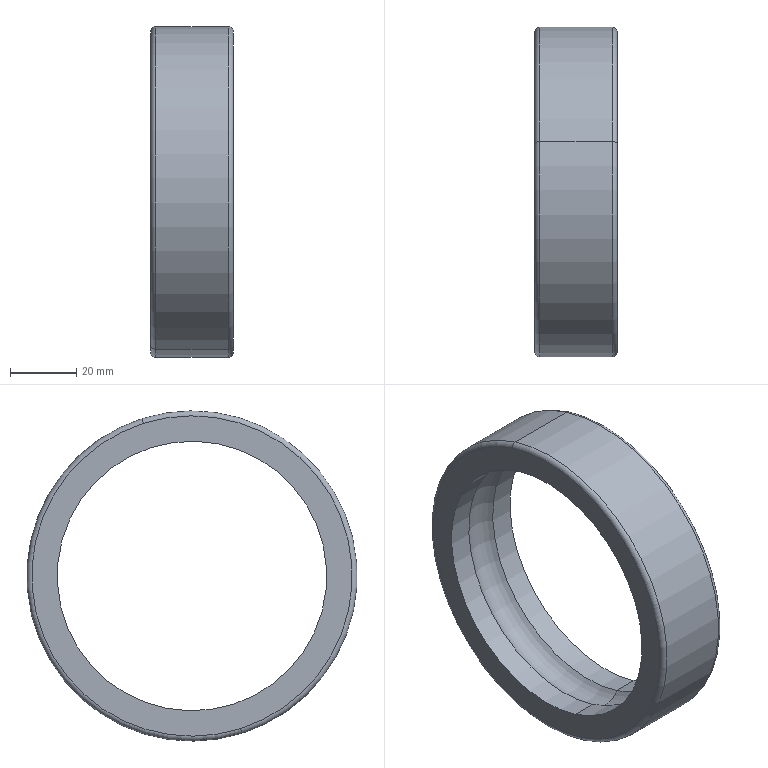Component | SolidWorks | UpperHousingAssembly-1_WormAxisAssembly-1_DeepGrooveBallBearing6309-1_BearingOuterRing-1 | 1 solid | 14 faces | box 25 x 100 x 100 mm | volume 61028 mm3 | torus 6 | cylinder 6 | plane 2 | commonest cylinder face diameters 81.6 x4 100 x2
build123d program:
from build123d import *

# Parameters (mm, degrees)
FILLET1_R = 1.5


with BuildPart() as part:
    # Sketch1 → Revolve1 (revolve)
    with BuildSketch(Plane.XY, mode=Mode.PRIVATE) as revolve1_sk:
        with BuildLine():
            Line((5.121, 40.8), (12.5, 40.8))
            Line((12.5, 40.8), (12.5, 50))
            Line((12.5, 50), (-12.5, 50))
            Line((-12.5, 50), (-12.5, 40.8))
            Line((-12.5, 40.8), (-5.121, 40.8))
            ThreePointArc((-5.121, 40.8), (0, 43.1), (5.121, 40.8))
        make_face()
    revolve(revolve1_sk.sketch.rotate(Axis((-5.851, 0, 0), (1, 0, 0)), 90), axis=Axis((-5.851, 0, 0), (1, 0, 0)))

    # Fillet1
    fillet1_edges = [part.edges().sort_by_distance(p)[0] for p in [
        (-12.5, 0, -50),
        (12.5, 0, -50),
    ]]
    fillet(fillet1_edges, radius=FILLET1_R)


solid = part.part

# Placed as in the assembly
solid = solid.moved(Location((1019.077, 1408.591, 1694.217), (0, 0, 0)))
STEP:
#1=CARTESIAN_POINT('',(40.613,54.879,64.881));
#2=VERTEX_POINT('',#1);
#3=CARTESIAN_POINT('',(40.613,56.034,68.522));
#4=VERTEX_POINT('',#3);
#5=CARTESIAN_POINT('',(40.613,55.456,66.701));
#6=DIRECTION('',(1.,0.,0.));
#7=DIRECTION('',(0.,0.3024,0.9532));
#8=AXIS2_PLACEMENT_3D('',#5,#6,#7);
#9=CIRCLE('',#8,1.909);
#10=EDGE_CURVE('',#2,#4,#9,.T.);
#11=ORIENTED_EDGE('',*,*,#10,.F.);
#12=CARTESIAN_POINT('',(40.554,54.861,64.825));
#13=VERTEX_POINT('',#12);
#14=CARTESIAN_POINT('',(40.554,54.879,64.881));
#15=DIRECTION('',(0.,0.9532,-0.3024));
#16=DIRECTION('',(0.,0.3024,0.9532));
#17=AXIS2_PLACEMENT_3D('',#14,#15,#16);
#18=CIRCLE('',#17,0.05906);
#19=EDGE_CURVE('',#2,#13,#18,.T.);
#20=ORIENTED_EDGE('',*,*,#19,.T.);
#21=CARTESIAN_POINT('',(40.554,56.052,68.578));
#22=VERTEX_POINT('',#21);
#23=CARTESIAN_POINT('',(40.554,55.456,66.701));
#24=DIRECTION('',(-1.,0.,0.));
#25=DIRECTION('',(0.,0.3024,0.9532));
#26=AXIS2_PLACEMENT_3D('',#23,#24,#25);
#27=CIRCLE('',#26,1.969);
#28=EDGE_CURVE('',#22,#13,#27,.T.);
#29=ORIENTED_EDGE('',*,*,#28,.F.);
#30=CARTESIAN_POINT('',(40.554,56.034,68.522));
#31=DIRECTION('',(0.,-0.9532,0.3024));
#32=DIRECTION('',(0.,-0.3024,-0.9532));
#33=AXIS2_PLACEMENT_3D('',#30,#31,#32);
#34=CIRCLE('',#33,0.05906);
#35=EDGE_CURVE('',#4,#22,#34,.T.);
#36=ORIENTED_EDGE('',*,*,#35,.F.);
#37=EDGE_LOOP('',(#11,#20,#29,#36));
#38=FACE_OUTER_BOUND('',#37,.T.);
#39=CARTESIAN_POINT('',(40.554,55.456,66.701));
#40=DIRECTION('',(-1.,0.,0.));
#41=DIRECTION('',(0.,0.3024,0.9532));
#42=AXIS2_PLACEMENT_3D('',#39,#40,#41);
#43=TOROIDAL_SURFACE('',#42,1.909,0.05906);
#44=ADVANCED_FACE('',(#38),#43,.T.);
#45=CARTESIAN_POINT('',(39.629,56.034,68.522));
#46=VERTEX_POINT('',#45);
#47=CARTESIAN_POINT('',(39.629,54.879,64.881));
#48=VERTEX_POINT('',#47);
#49=CARTESIAN_POINT('',(39.629,55.456,66.701));
#50=DIRECTION('',(-1.,0.,0.));
#51=DIRECTION('',(0.,-0.3024,-0.9532));
#52=AXIS2_PLACEMENT_3D('',#49,#50,#51);
#53=CIRCLE('',#52,1.909);
#54=EDGE_CURVE('',#46,#48,#53,.T.);
#55=ORIENTED_EDGE('',*,*,#54,.F.);
#56=CARTESIAN_POINT('',(39.688,56.052,68.578));
#57=VERTEX_POINT('',#56);
#58=CARTESIAN_POINT('',(39.688,56.034,68.522));
#59=DIRECTION('',(0.,0.9532,-0.3024));
#60=DIRECTION('',(0.,0.3024,0.9532));
#61=AXIS2_PLACEMENT_3D('',#58,#59,#60);
#62=CIRCLE('',#61,0.05906);
#63=EDGE_CURVE('',#46,#57,#62,.T.);
#64=ORIENTED_EDGE('',*,*,#63,.T.);
#65=CARTESIAN_POINT('',(39.688,54.861,64.825));
#66=VERTEX_POINT('',#65);
#67=CARTESIAN_POINT('',(39.688,55.456,66.701));
#68=DIRECTION('',(1.,0.,0.));
#69=DIRECTION('',(0.,-0.3024,-0.9532));
#70=AXIS2_PLACEMENT_3D('',#67,#68,#69);
#71=CIRCLE('',#70,1.969);
#72=EDGE_CURVE('',#66,#57,#71,.T.);
#73=ORIENTED_EDGE('',*,*,#72,.F.);
#74=CARTESIAN_POINT('',(39.688,54.879,64.881));
#75=DIRECTION('',(0.,-0.9532,0.3024));
#76=DIRECTION('',(0.,-0.3024,-0.9532));
#77=AXIS2_PLACEMENT_3D('',#74,#75,#76);
#78=CIRCLE('',#77,0.05906);
#79=EDGE_CURVE('',#48,#66,#78,.T.);
#80=ORIENTED_EDGE('',*,*,#79,.F.);
#81=EDGE_LOOP('',(#55,#64,#73,#80));
#82=FACE_OUTER_BOUND('',#81,.T.);
#83=CARTESIAN_POINT('',(39.688,55.456,66.701));
#84=DIRECTION('',(1.,0.,0.));
#85=DIRECTION('',(0.,-0.3024,-0.9532));
#86=AXIS2_PLACEMENT_3D('',#83,#84,#85);
#87=TOROIDAL_SURFACE('',#86,1.909,0.05906);
#88=ADVANCED_FACE('',(#82),#87,.T.);
#89=CARTESIAN_POINT('',(40.613,54.971,65.17));
#90=VERTEX_POINT('',#89);
#91=CARTESIAN_POINT('',(40.613,55.942,68.233));
#92=VERTEX_POINT('',#91);
#93=CARTESIAN_POINT('',(40.613,55.456,66.701));
#94=DIRECTION('',(-1.,0.,0.));
#95=DIRECTION('',(0.,0.3024,0.9532));
#96=AXIS2_PLACEMENT_3D('',#93,#94,#95);
#97=CIRCLE('',#96,1.606);
#98=EDGE_CURVE('',#90,#92,#97,.T.);
#99=ORIENTED_EDGE('',*,*,#98,.F.);
#100=CARTESIAN_POINT('',(40.323,54.971,65.17));
#101=VERTEX_POINT('',#100);
#102=CARTESIAN_POINT('',(39.891,54.971,65.17));
#103=DIRECTION('',(-1.,0.,0.));
#104=VECTOR('',#103,39.37);
#105=LINE('',#102,#104);
#106=EDGE_CURVE('',#90,#101,#105,.T.);
#107=ORIENTED_EDGE('',*,*,#106,.T.);
#108=CARTESIAN_POINT('',(40.323,55.942,68.233));
#109=VERTEX_POINT('',#108);
#110=CARTESIAN_POINT('',(40.323,55.456,66.701));
#111=DIRECTION('',(-1.,0.,0.));
#112=DIRECTION('',(0.,0.3024,0.9532));
#113=AXIS2_PLACEMENT_3D('',#110,#111,#112);
#114=CIRCLE('',#113,1.606);
#115=EDGE_CURVE('',#101,#109,#114,.T.);
#116=ORIENTED_EDGE('',*,*,#115,.T.);
#117=CARTESIAN_POINT('',(39.891,55.942,68.233));
#118=DIRECTION('',(-1.,0.,0.));
#119=VECTOR('',#118,39.37);
#120=LINE('',#117,#119);
#121=EDGE_CURVE('',#92,#109,#120,.T.);
#122=ORIENTED_EDGE('',*,*,#121,.F.);
#123=EDGE_LOOP('',(#99,#107,#116,#122));
#124=FACE_OUTER_BOUND('',#123,.T.);
#125=CARTESIAN_POINT('',(39.891,55.456,66.701));
#126=DIRECTION('',(-1.,0.,0.));
#127=DIRECTION('',(0.,0.3024,0.9532));
#128=AXIS2_PLACEMENT_3D('',#125,#126,#127);
#129=CYLINDRICAL_SURFACE('',#128,1.606);
#130=ADVANCED_FACE('',(#124),#129,.F.);
#131=ORIENTED_EDGE('',*,*,#115,.F.);
#132=CARTESIAN_POINT('',(39.92,54.971,65.17));
#133=VERTEX_POINT('',#132);
#134=CARTESIAN_POINT('',(40.121,55.025,65.341));
#135=DIRECTION('',(0.,0.9532,-0.3024));
#136=DIRECTION('',(0.,0.3024,0.9532));
#137=AXIS2_PLACEMENT_3D('',#134,#135,#136);
#138=CIRCLE('',#137,0.2697);
#139=EDGE_CURVE('',#101,#133,#138,.T.);
#140=ORIENTED_EDGE('',*,*,#139,.T.);
#141=CARTESIAN_POINT('',(39.92,55.942,68.233));
#142=VERTEX_POINT('',#141);
#143=CARTESIAN_POINT('',(39.92,55.456,66.701));
#144=DIRECTION('',(-1.,0.,0.));
#145=DIRECTION('',(0.,0.3024,0.9532));
#146=AXIS2_PLACEMENT_3D('',#143,#144,#145);
#147=CIRCLE('',#146,1.606);
#148=EDGE_CURVE('',#133,#142,#147,.T.);
#149=ORIENTED_EDGE('',*,*,#148,.T.);
#150=CARTESIAN_POINT('',(40.121,55.888,68.062));
#151=DIRECTION('',(0.,-0.9532,0.3024));
#152=DIRECTION('',(0.,-0.3024,-0.9532));
#153=AXIS2_PLACEMENT_3D('',#150,#151,#152);
#154=CIRCLE('',#153,0.2697);
#155=EDGE_CURVE('',#109,#142,#154,.T.);
#156=ORIENTED_EDGE('',*,*,#155,.F.);
#157=EDGE_LOOP('',(#131,#140,#149,#156));
#158=FACE_OUTER_BOUND('',#157,.T.);
#159=CARTESIAN_POINT('',(40.121,55.456,66.701));
#160=DIRECTION('',(-1.,0.,0.));
#161=DIRECTION('',(0.,0.3024,0.9532));
#162=AXIS2_PLACEMENT_3D('',#159,#160,#161);
#163=TOROIDAL_SURFACE('',#162,1.427,0.2697);
#164=ADVANCED_FACE('',(#158),#163,.F.);
#165=ORIENTED_EDGE('',*,*,#148,.F.);
#166=CARTESIAN_POINT('',(39.629,54.971,65.17));
#167=VERTEX_POINT('',#166);
#168=CARTESIAN_POINT('',(39.891,54.971,65.17));
#169=DIRECTION('',(-1.,0.,0.));
#170=VECTOR('',#169,39.37);
#171=LINE('',#168,#170);
#172=EDGE_CURVE('',#133,#167,#171,.T.);
#173=ORIENTED_EDGE('',*,*,#172,.T.);
#174=CARTESIAN_POINT('',(39.629,55.942,68.233));
#175=VERTEX_POINT('',#174);
#176=CARTESIAN_POINT('',(39.629,55.456,66.701));
#177=DIRECTION('',(-1.,0.,0.));
#178=DIRECTION('',(0.,0.3024,0.9532));
#179=AXIS2_PLACEMENT_3D('',#176,#177,#178);
#180=CIRCLE('',#179,1.606);
#181=EDGE_CURVE('',#167,#175,#180,.T.);
#182=ORIENTED_EDGE('',*,*,#181,.T.);
#183=CARTESIAN_POINT('',(39.891,55.942,68.233));
#184=DIRECTION('',(-1.,0.,0.));
#185=VECTOR('',#184,39.37);
#186=LINE('',#183,#185);
#187=EDGE_CURVE('',#142,#175,#186,.T.);
#188=ORIENTED_EDGE('',*,*,#187,.F.);
#189=EDGE_LOOP('',(#165,#173,#182,#188));
#190=FACE_OUTER_BOUND('',#189,.T.);
#191=CARTESIAN_POINT('',(39.891,55.456,66.701));
#192=DIRECTION('',(-1.,0.,0.));
#193=DIRECTION('',(0.,0.3024,0.9532));
#194=AXIS2_PLACEMENT_3D('',#191,#192,#193);
#195=CYLINDRICAL_SURFACE('',#194,1.606);
#196=ADVANCED_FACE('',(#190),#195,.F.);
#197=ORIENTED_EDGE('',*,*,#28,.T.);
#198=CARTESIAN_POINT('',(39.891,54.861,64.825));
#199=DIRECTION('',(-1.,0.,0.));
#200=VECTOR('',#199,39.37);
#201=LINE('',#198,#200);
#202=EDGE_CURVE('',#13,#66,#201,.T.);
#203=ORIENTED_EDGE('',*,*,#202,.T.);
#204=ORIENTED_EDGE('',*,*,#72,.T.);
#205=CARTESIAN_POINT('',(39.891,56.052,68.578));
#206=DIRECTION('',(-1.,0.,0.));
#207=VECTOR('',#206,39.37);
#208=LINE('',#205,#207);
#209=EDGE_CURVE('',#22,#57,#208,.T.);
#210=ORIENTED_EDGE('',*,*,#209,.F.);
#211=EDGE_LOOP('',(#197,#203,#204,#210));
#212=FACE_OUTER_BOUND('',#211,.T.);
#213=CARTESIAN_POINT('',(39.891,55.456,66.701));
#214=DIRECTION('',(-1.,0.,0.));
#215=DIRECTION('',(0.,0.3024,0.9532));
#216=AXIS2_PLACEMENT_3D('',#213,#214,#215);
#217=CYLINDRICAL_SURFACE('',#216,1.969);
#218=ADVANCED_FACE('',(#212),#217,.T.);
#219=CARTESIAN_POINT('',(40.613,55.456,66.701));
#220=DIRECTION('',(1.,0.,0.));
#221=DIRECTION('',(0.,0.3024,0.9532));
#222=AXIS2_PLACEMENT_3D('',#219,#220,#221);
#223=CIRCLE('',#222,1.909);
#224=EDGE_CURVE('',#4,#2,#223,.T.);
#225=ORIENTED_EDGE('',*,*,#224,.T.);
#226=ORIENTED_EDGE('',*,*,#10,.T.);
#227=EDGE_LOOP('',(#225,#226));
#228=FACE_OUTER_BOUND('',#227,.T.);
#229=CARTESIAN_POINT('',(40.613,55.456,66.701));
#230=DIRECTION('',(-1.,0.,0.));
#231=DIRECTION('',(0.,0.3024,0.9532));
#232=AXIS2_PLACEMENT_3D('',#229,#230,#231);
#233=CIRCLE('',#232,1.606);
#234=EDGE_CURVE('',#92,#90,#233,.T.);
#235=ORIENTED_EDGE('',*,*,#234,.T.);
#236=ORIENTED_EDGE('',*,*,#98,.T.);
#237=EDGE_LOOP('',(#235,#236));
#238=FACE_BOUND('',#237,.T.);
#239=CARTESIAN_POINT('',(40.613,57.333,66.106));
#240=DIRECTION('',(-1.,0.,0.));
#241=DIRECTION('',(0.,0.3024,0.9532));
#242=AXIS2_PLACEMENT_3D('',#239,#240,#241);
#243=PLANE('',#242);
#244=ADVANCED_FACE('',(#228,#238),#243,.F.);
#245=ORIENTED_EDGE('',*,*,#202,.F.);
#246=CARTESIAN_POINT('',(40.554,55.456,66.701));
#247=DIRECTION('',(-1.,0.,0.));
#248=DIRECTION('',(0.,0.3024,0.9532));
#249=AXIS2_PLACEMENT_3D('',#246,#247,#248);
#250=CIRCLE('',#249,1.969);
#251=EDGE_CURVE('',#13,#22,#250,.T.);
#252=ORIENTED_EDGE('',*,*,#251,.T.);
#253=ORIENTED_EDGE('',*,*,#209,.T.);
#254=CARTESIAN_POINT('',(39.688,55.456,66.701));
#255=DIRECTION('',(1.,0.,0.));
#256=DIRECTION('',(0.,-0.3024,-0.9532));
#257=AXIS2_PLACEMENT_3D('',#254,#255,#256);
#258=CIRCLE('',#257,1.969);
#259=EDGE_CURVE('',#57,#66,#258,.T.);
#260=ORIENTED_EDGE('',*,*,#259,.T.);
#261=EDGE_LOOP('',(#245,#252,#253,#260));
#262=FACE_OUTER_BOUND('',#261,.T.);
#263=CARTESIAN_POINT('',(39.891,55.456,66.701));
#264=DIRECTION('',(-1.,0.,0.));
#265=DIRECTION('',(0.,0.3024,0.9532));
#266=AXIS2_PLACEMENT_3D('',#263,#264,#265);
#267=CYLINDRICAL_SURFACE('',#266,1.969);
#268=ADVANCED_FACE('',(#262),#267,.T.);
#269=CARTESIAN_POINT('',(39.629,55.456,66.701));
#270=DIRECTION('',(-1.,0.,0.));
#271=DIRECTION('',(0.,-0.3024,-0.9532));
#272=AXIS2_PLACEMENT_3D('',#269,#270,#271);
#273=CIRCLE('',#272,1.909);
#274=EDGE_CURVE('',#48,#46,#273,.T.);
#275=ORIENTED_EDGE('',*,*,#274,.T.);
#276=ORIENTED_EDGE('',*,*,#54,.T.);
#277=EDGE_LOOP('',(#275,#276));
#278=FACE_OUTER_BOUND('',#277,.T.);
#279=CARTESIAN_POINT('',(39.629,55.456,66.701));
#280=DIRECTION('',(-1.,0.,0.));
#281=DIRECTION('',(0.,0.3024,0.9532));
#282=AXIS2_PLACEMENT_3D('',#279,#280,#281);
#283=CIRCLE('',#282,1.606);
#284=EDGE_CURVE('',#175,#167,#283,.T.);
#285=ORIENTED_EDGE('',*,*,#284,.F.);
#286=ORIENTED_EDGE('',*,*,#181,.F.);
#287=EDGE_LOOP('',(#285,#286));
#288=FACE_BOUND('',#287,.T.);
#289=CARTESIAN_POINT('',(39.629,57.333,66.106));
#290=DIRECTION('',(1.,0.,0.));
#291=DIRECTION('',(0.,-0.3024,-0.9532));
#292=AXIS2_PLACEMENT_3D('',#289,#290,#291);
#293=PLANE('',#292);
#294=ADVANCED_FACE('',(#278,#288),#293,.F.);
#295=ORIENTED_EDGE('',*,*,#172,.F.);
#296=CARTESIAN_POINT('',(39.92,55.456,66.701));
#297=DIRECTION('',(-1.,0.,0.));
#298=DIRECTION('',(0.,0.3024,0.9532));
#299=AXIS2_PLACEMENT_3D('',#296,#297,#298);
#300=CIRCLE('',#299,1.606);
#301=EDGE_CURVE('',#142,#133,#300,.T.);
#302=ORIENTED_EDGE('',*,*,#301,.F.);
#303=ORIENTED_EDGE('',*,*,#187,.T.);
#304=ORIENTED_EDGE('',*,*,#284,.T.);
#305=EDGE_LOOP('',(#295,#302,#303,#304));
#306=FACE_OUTER_BOUND('',#305,.T.);
#307=CARTESIAN_POINT('',(39.891,55.456,66.701));
#308=DIRECTION('',(-1.,0.,0.));
#309=DIRECTION('',(0.,0.3024,0.9532));
#310=AXIS2_PLACEMENT_3D('',#307,#308,#309);
#311=CYLINDRICAL_SURFACE('',#310,1.606);
#312=ADVANCED_FACE('',(#306),#311,.F.);
#313=ORIENTED_EDGE('',*,*,#139,.F.);
#314=CARTESIAN_POINT('',(40.323,55.456,66.701));
#315=DIRECTION('',(-1.,0.,0.));
#316=DIRECTION('',(0.,0.3024,0.9532));
#317=AXIS2_PLACEMENT_3D('',#314,#315,#316);
#318=CIRCLE('',#317,1.606);
#319=EDGE_CURVE('',#109,#101,#318,.T.);
#320=ORIENTED_EDGE('',*,*,#319,.F.);
#321=ORIENTED_EDGE('',*,*,#155,.T.);
#322=ORIENTED_EDGE('',*,*,#301,.T.);
#323=EDGE_LOOP('',(#313,#320,#321,#322));
#324=FACE_OUTER_BOUND('',#323,.T.);
#325=CARTESIAN_POINT('',(40.121,55.456,66.701));
#326=DIRECTION('',(-1.,0.,0.));
#327=DIRECTION('',(0.,0.3024,0.9532));
#328=AXIS2_PLACEMENT_3D('',#325,#326,#327);
#329=TOROIDAL_SURFACE('',#328,1.427,0.2697);
#330=ADVANCED_FACE('',(#324),#329,.F.);
#331=ORIENTED_EDGE('',*,*,#106,.F.);
#332=ORIENTED_EDGE('',*,*,#234,.F.);
#333=ORIENTED_EDGE('',*,*,#121,.T.);
#334=ORIENTED_EDGE('',*,*,#319,.T.);
#335=EDGE_LOOP('',(#331,#332,#333,#334));
#336=FACE_OUTER_BOUND('',#335,.T.);
#337=CARTESIAN_POINT('',(39.891,55.456,66.701));
#338=DIRECTION('',(-1.,0.,0.));
#339=DIRECTION('',(0.,0.3024,0.9532));
#340=AXIS2_PLACEMENT_3D('',#337,#338,#339);
#341=CYLINDRICAL_SURFACE('',#340,1.606);
#342=ADVANCED_FACE('',(#336),#341,.F.);
#343=ORIENTED_EDGE('',*,*,#63,.F.);
#344=ORIENTED_EDGE('',*,*,#274,.F.);
#345=ORIENTED_EDGE('',*,*,#79,.T.);
#346=ORIENTED_EDGE('',*,*,#259,.F.);
#347=EDGE_LOOP('',(#343,#344,#345,#346));
#348=FACE_OUTER_BOUND('',#347,.T.);
#349=CARTESIAN_POINT('',(39.688,55.456,66.701));
#350=DIRECTION('',(1.,0.,0.));
#351=DIRECTION('',(0.,-0.3024,-0.9532));
#352=AXIS2_PLACEMENT_3D('',#349,#350,#351);
#353=TOROIDAL_SURFACE('',#352,1.909,0.05906);
#354=ADVANCED_FACE('',(#348),#353,.T.);
#355=ORIENTED_EDGE('',*,*,#19,.F.);
#356=ORIENTED_EDGE('',*,*,#224,.F.);
#357=ORIENTED_EDGE('',*,*,#35,.T.);
#358=ORIENTED_EDGE('',*,*,#251,.F.);
#359=EDGE_LOOP('',(#355,#356,#357,#358));
#360=FACE_OUTER_BOUND('',#359,.T.);
#361=CARTESIAN_POINT('',(40.554,55.456,66.701));
#362=DIRECTION('',(-1.,0.,0.));
#363=DIRECTION('',(0.,0.3024,0.9532));
#364=AXIS2_PLACEMENT_3D('',#361,#362,#363);
#365=TOROIDAL_SURFACE('',#364,1.909,0.05906);
#366=ADVANCED_FACE('',(#360),#365,.T.);
#367=CLOSED_SHELL('',(#44,#88,#130,#164,#196,#218,#244,#268,#294,#312,#330,#342,#354,#366));
#368=MANIFOLD_SOLID_BREP('',#367);
#369=CARTESIAN_POINT('',(0.,0.,0.));
#370=DIRECTION('',(0.,0.,1.));
#371=DIRECTION('',(1.,0.,0.));
#372=AXIS2_PLACEMENT_3D('',#369,#370,#371);
#373=(LENGTH_UNIT()NAMED_UNIT(*)SI_UNIT($,.METRE.));
#374=LENGTH_MEASURE_WITH_UNIT(LENGTH_MEASURE(0.0254),#373);
#375=DIMENSIONAL_EXPONENTS(1.,0.,0.,0.,0.,0.,0.);
#376=(CONVERSION_BASED_UNIT('',#374)LENGTH_UNIT()NAMED_UNIT(#375));
#377=UNCERTAINTY_MEASURE_WITH_UNIT(LENGTH_MEASURE(0.00001),#376,'','');
#378=(NAMED_UNIT(*)PLANE_ANGLE_UNIT()SI_UNIT($,.RADIAN.));
#379=(NAMED_UNIT(*)SI_UNIT($,.STERADIAN.)SOLID_ANGLE_UNIT());
#380=(GEOMETRIC_REPRESENTATION_CONTEXT(3)GLOBAL_UNCERTAINTY_ASSIGNED_CONTEXT((#377))GLOBAL_UNIT_ASSIGNED_CONTEXT((#376,#378,#379))REPRESENTATION_CONTEXT('',''));
#381=ADVANCED_BREP_SHAPE_REPRESENTATION('',(#368,#372),#380);
#382=COLOUR_RGB('',0.7922,0.8196,0.9333);
#383=FILL_AREA_STYLE_COLOUR('',#382);
#384=FILL_AREA_STYLE('',(#383));
#385=SURFACE_STYLE_FILL_AREA(#384);
#386=SURFACE_SIDE_STYLE('',(#385));
#387=SURFACE_STYLE_USAGE(.BOTH.,#386);
#388=PRESENTATION_STYLE_ASSIGNMENT((#387));
#389=STYLED_ITEM('',(#388),#368);
#390=(LENGTH_UNIT()NAMED_UNIT(*)SI_UNIT($,.METRE.));
#391=LENGTH_MEASURE_WITH_UNIT(LENGTH_MEASURE(0.0254),#390);
#392=DIMENSIONAL_EXPONENTS(1.,0.,0.,0.,0.,0.,0.);
#393=(CONVERSION_BASED_UNIT('',#391)LENGTH_UNIT()NAMED_UNIT(#392));
#394=UNCERTAINTY_MEASURE_WITH_UNIT(LENGTH_MEASURE(0.00001),#393,'','');
#395=(NAMED_UNIT(*)PLANE_ANGLE_UNIT()SI_UNIT($,.RADIAN.));
#396=(NAMED_UNIT(*)SI_UNIT($,.STERADIAN.)SOLID_ANGLE_UNIT());
#397=(GEOMETRIC_REPRESENTATION_CONTEXT(3)GLOBAL_UNCERTAINTY_ASSIGNED_CONTEXT((#394))GLOBAL_UNIT_ASSIGNED_CONTEXT((#393,#395,#396))REPRESENTATION_CONTEXT('',''));
#398=MECHANICAL_DESIGN_GEOMETRIC_PRESENTATION_REPRESENTATION('',(#389),#397);
#399=PRESENTATION_LAYER_ASSIGNMENT('','',(#389));